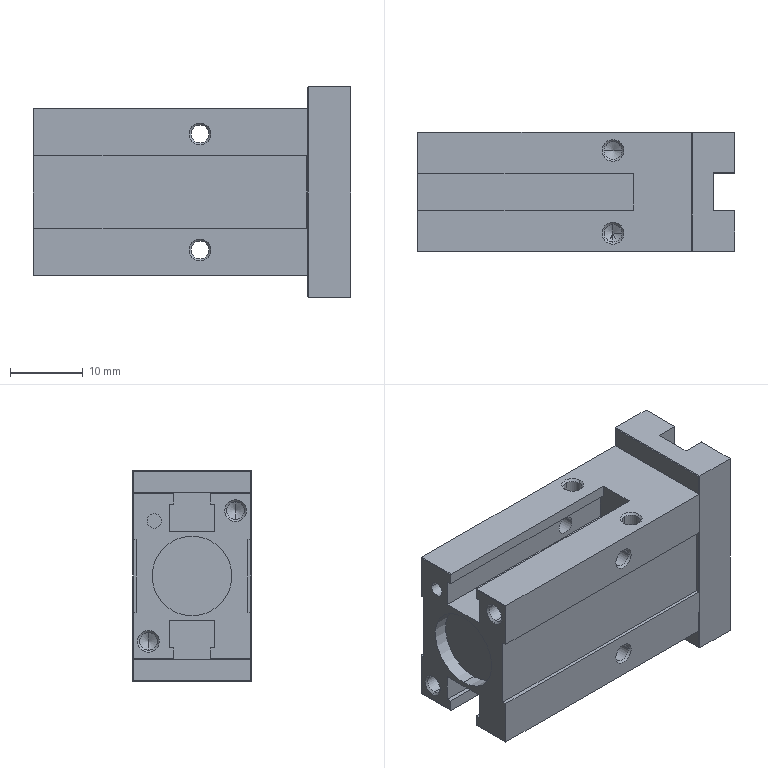Component | SolidWorks | MHZ2-10D-1_CopyBodyA_MHZ2-10D(11.2)-1 | 1 solid | 111 faces | volume 13905 mm3 | plane 58 | cone 29 | cylinder 24 | commonest cylinder face diameters 2.46 x20 11 x2 2 x2